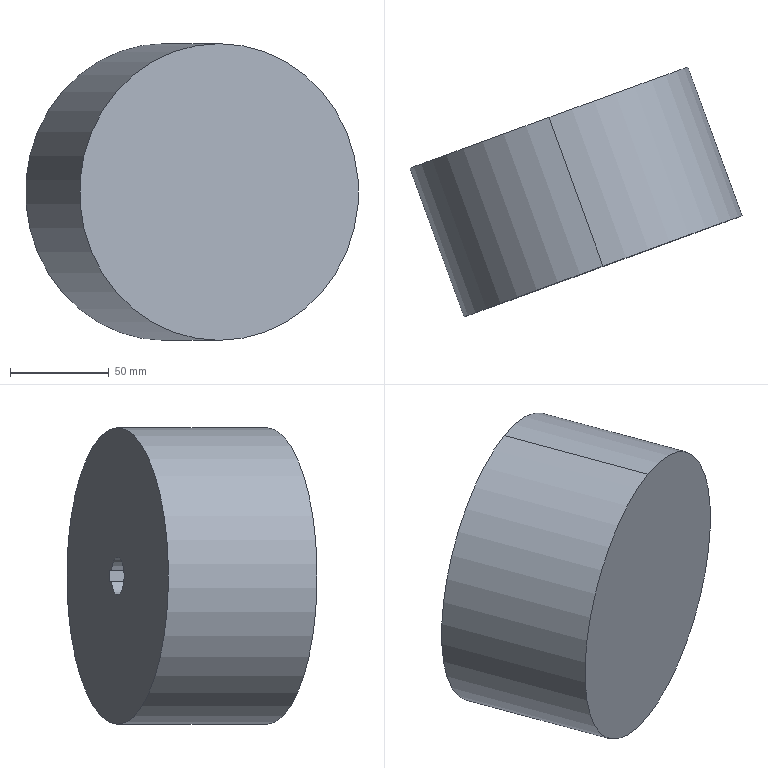Component | SolidWorks | 03-03BallDeliveryWheel-1 | 1 solid | 11 faces | box 168.32 x 126.48 x 150 mm | volume 1410704 mm3 | plane 6 | cylinder 5 | commonest cylinder face diameters 19 x3 150 x2
build123d program:
from build123d import *

# Parameters (mm, degrees)
SKETCH1_2_R         = 75
BOSS_EXTRUDE1_DEPTH = 80
CUT_EXTRUDE1_DEPTH  = 10


with BuildPart() as part:
    # Sketch1_2 → Boss-Extrude1 (new body)
    with BuildSketch(Plane(origin=(0, 0, 0), x_dir=(1, 0, 0), z_dir=(0, 1, 0))):
        with Locations(Location((0, 0, 0), (0, 0, 270))):
            Circle(SKETCH1_2_R)
    extrude(amount=BOSS_EXTRUDE1_DEPTH)

    # Sketch1 → Cut-Extrude1 (cut)
    with BuildSketch(Plane(origin=(0, 80, 0), x_dir=(1, 0, 0), z_dir=(0, 1, 0))):
        with BuildLine():
            Line((9.014, -3), (12.3, -3))
            Line((12.3, -3), (12.3, 3))
            Line((12.3, 3), (9.014, 3))
            ThreePointArc((9.014, 3), (-9.5, 0), (9.014, -3))
        make_face()
    extrude(amount=-CUT_EXTRUDE1_DEPTH, mode=Mode.SUBTRACT)


solid = part.part

# Placed as in the assembly
solid = solid.moved(Location((285.217, 218.335, 175), (0, 0, 20)))
STEP:
#1=COLOUR_RGB('',0.7922,0.8196,0.9333);
#2=FILL_AREA_STYLE_COLOUR('',#1);
#3=FILL_AREA_STYLE('',(#2));
#4=SURFACE_STYLE_FILL_AREA(#3);
#5=SURFACE_SIDE_STYLE('',(#4));
#6=SURFACE_STYLE_USAGE(.BOTH.,#5);
#7=PRESENTATION_STYLE_ASSIGNMENT((#6));
#8=CARTESIAN_POINT('',(10.286,11.186,6.516));
#9=VERTEX_POINT('',#8);
#10=CARTESIAN_POINT('',(10.286,11.186,7.264));
#11=VERTEX_POINT('',#10);
#12=CARTESIAN_POINT('',(10.286,11.186,6.89));
#13=DIRECTION('',(-0.342,0.9397,0.));
#14=DIRECTION('',(0.,0.,1.));
#15=AXIS2_PLACEMENT_3D('',#12,#13,#14);
#16=CIRCLE('',#15,0.374);
#17=EDGE_CURVE('',#9,#11,#16,.T.);
#18=ORIENTED_EDGE('',*,*,#17,.F.);
#19=CARTESIAN_POINT('',(10.152,11.556,6.516));
#20=VERTEX_POINT('',#19);
#21=CARTESIAN_POINT('',(10.286,11.186,6.516));
#22=DIRECTION('',(-0.342,0.9397,0.));
#23=VECTOR('',#22,39.37);
#24=LINE('',#21,#23);
#25=EDGE_CURVE('',#9,#20,#24,.T.);
#26=ORIENTED_EDGE('',*,*,#25,.T.);
#27=CARTESIAN_POINT('',(10.152,11.556,7.264));
#28=VERTEX_POINT('',#27);
#29=CARTESIAN_POINT('',(10.152,11.556,6.89));
#30=DIRECTION('',(-0.342,0.9397,0.));
#31=DIRECTION('',(0.,0.,1.));
#32=AXIS2_PLACEMENT_3D('',#29,#30,#31);
#33=CIRCLE('',#32,0.374);
#34=EDGE_CURVE('',#20,#28,#33,.T.);
#35=ORIENTED_EDGE('',*,*,#34,.T.);
#36=CARTESIAN_POINT('',(10.286,11.186,7.264));
#37=DIRECTION('',(-0.342,0.9397,0.));
#38=VECTOR('',#37,39.37);
#39=LINE('',#36,#38);
#40=EDGE_CURVE('',#11,#28,#39,.T.);
#41=ORIENTED_EDGE('',*,*,#40,.F.);
#42=EDGE_LOOP('',(#18,#26,#35,#41));
#43=FACE_OUTER_BOUND('',#42,.T.);
#44=CARTESIAN_POINT('',(10.286,11.186,6.89));
#45=DIRECTION('',(-0.342,0.9397,0.));
#46=DIRECTION('',(0.,0.,1.));
#47=AXIS2_PLACEMENT_3D('',#44,#45,#46);
#48=CYLINDRICAL_SURFACE('',#47,0.374);
#49=ADVANCED_FACE('',(#43),#48,.F.);
#50=CARTESIAN_POINT('',(10.62,11.307,7.008));
#51=VERTEX_POINT('',#50);
#52=CARTESIAN_POINT('',(10.286,11.186,6.89));
#53=DIRECTION('',(-0.342,0.9397,0.));
#54=DIRECTION('',(0.,0.,1.));
#55=AXIS2_PLACEMENT_3D('',#52,#53,#54);
#56=CIRCLE('',#55,0.374);
#57=EDGE_CURVE('',#11,#51,#56,.T.);
#58=ORIENTED_EDGE('',*,*,#57,.F.);
#59=ORIENTED_EDGE('',*,*,#40,.T.);
#60=CARTESIAN_POINT('',(10.485,11.677,7.008));
#61=VERTEX_POINT('',#60);
#62=CARTESIAN_POINT('',(10.152,11.556,6.89));
#63=DIRECTION('',(-0.342,0.9397,0.));
#64=DIRECTION('',(0.,0.,1.));
#65=AXIS2_PLACEMENT_3D('',#62,#63,#64);
#66=CIRCLE('',#65,0.374);
#67=EDGE_CURVE('',#28,#61,#66,.T.);
#68=ORIENTED_EDGE('',*,*,#67,.T.);
#69=CARTESIAN_POINT('',(10.62,11.307,7.008));
#70=DIRECTION('',(-0.342,0.9397,0.));
#71=VECTOR('',#70,39.37);
#72=LINE('',#69,#71);
#73=EDGE_CURVE('',#51,#61,#72,.T.);
#74=ORIENTED_EDGE('',*,*,#73,.F.);
#75=EDGE_LOOP('',(#58,#59,#68,#74));
#76=FACE_OUTER_BOUND('',#75,.T.);
#77=CARTESIAN_POINT('',(10.286,11.186,6.89));
#78=DIRECTION('',(-0.342,0.9397,0.));
#79=DIRECTION('',(0.,0.,1.));
#80=AXIS2_PLACEMENT_3D('',#77,#78,#79);
#81=CYLINDRICAL_SURFACE('',#80,0.374);
#82=ADVANCED_FACE('',(#76),#81,.F.);
#83=CARTESIAN_POINT('',(10.152,11.556,9.843));
#84=VERTEX_POINT('',#83);
#85=CARTESIAN_POINT('',(10.152,11.556,3.937));
#86=VERTEX_POINT('',#85);
#87=CARTESIAN_POINT('',(10.152,11.556,6.89));
#88=DIRECTION('',(-0.342,0.9397,0.));
#89=DIRECTION('',(0.,0.,1.));
#90=AXIS2_PLACEMENT_3D('',#87,#88,#89);
#91=CIRCLE('',#90,2.953);
#92=EDGE_CURVE('',#84,#86,#91,.T.);
#93=ORIENTED_EDGE('',*,*,#92,.F.);
#94=CARTESIAN_POINT('',(11.229,8.596,9.843));
#95=VERTEX_POINT('',#94);
#96=CARTESIAN_POINT('',(10.152,11.556,9.843));
#97=DIRECTION('',(0.342,-0.9397,-0.));
#98=VECTOR('',#97,39.37);
#99=LINE('',#96,#98);
#100=EDGE_CURVE('',#84,#95,#99,.T.);
#101=ORIENTED_EDGE('',*,*,#100,.T.);
#102=CARTESIAN_POINT('',(11.229,8.596,3.937));
#103=VERTEX_POINT('',#102);
#104=CARTESIAN_POINT('',(11.229,8.596,6.89));
#105=DIRECTION('',(-0.342,0.9397,0.));
#106=DIRECTION('',(0.,0.,1.));
#107=AXIS2_PLACEMENT_3D('',#104,#105,#106);
#108=CIRCLE('',#107,2.953);
#109=EDGE_CURVE('',#95,#103,#108,.T.);
#110=ORIENTED_EDGE('',*,*,#109,.T.);
#111=CARTESIAN_POINT('',(10.152,11.556,3.937));
#112=DIRECTION('',(0.342,-0.9397,-0.));
#113=VECTOR('',#112,39.37);
#114=LINE('',#111,#113);
#115=EDGE_CURVE('',#86,#103,#114,.T.);
#116=ORIENTED_EDGE('',*,*,#115,.F.);
#117=EDGE_LOOP('',(#93,#101,#110,#116));
#118=FACE_OUTER_BOUND('',#117,.T.);
#119=CARTESIAN_POINT('',(10.152,11.556,6.89));
#120=DIRECTION('',(0.342,-0.9397,-0.));
#121=DIRECTION('',(0.,0.,-1.));
#122=AXIS2_PLACEMENT_3D('',#119,#120,#121);
#123=CYLINDRICAL_SURFACE('',#122,2.953);
#124=ADVANCED_FACE('',(#118),#123,.T.);
#125=ORIENTED_EDGE('',*,*,#100,.F.);
#126=CARTESIAN_POINT('',(10.152,11.556,6.89));
#127=DIRECTION('',(-0.342,0.9397,0.));
#128=DIRECTION('',(0.,0.,1.));
#129=AXIS2_PLACEMENT_3D('',#126,#127,#128);
#130=CIRCLE('',#129,2.953);
#131=EDGE_CURVE('',#86,#84,#130,.T.);
#132=ORIENTED_EDGE('',*,*,#131,.F.);
#133=ORIENTED_EDGE('',*,*,#115,.T.);
#134=CARTESIAN_POINT('',(11.229,8.596,6.89));
#135=DIRECTION('',(-0.342,0.9397,0.));
#136=DIRECTION('',(0.,0.,1.));
#137=AXIS2_PLACEMENT_3D('',#134,#135,#136);
#138=CIRCLE('',#137,2.953);
#139=EDGE_CURVE('',#103,#95,#138,.T.);
#140=ORIENTED_EDGE('',*,*,#139,.T.);
#141=EDGE_LOOP('',(#125,#132,#133,#140));
#142=FACE_OUTER_BOUND('',#141,.T.);
#143=CARTESIAN_POINT('',(10.152,11.556,6.89));
#144=DIRECTION('',(0.342,-0.9397,-0.));
#145=DIRECTION('',(0.,0.,-1.));
#146=AXIS2_PLACEMENT_3D('',#143,#144,#145);
#147=CYLINDRICAL_SURFACE('',#146,2.953);
#148=ADVANCED_FACE('',(#142),#147,.T.);
#149=CARTESIAN_POINT('',(10.485,11.677,6.772));
#150=VERTEX_POINT('',#149);
#151=CARTESIAN_POINT('',(10.152,11.556,6.89));
#152=DIRECTION('',(-0.342,0.9397,0.));
#153=DIRECTION('',(0.,0.,1.));
#154=AXIS2_PLACEMENT_3D('',#151,#152,#153);
#155=CIRCLE('',#154,0.374);
#156=EDGE_CURVE('',#150,#20,#155,.T.);
#157=ORIENTED_EDGE('',*,*,#156,.F.);
#158=CARTESIAN_POINT('',(10.607,11.721,6.772));
#159=VERTEX_POINT('',#158);
#160=CARTESIAN_POINT('',(10.607,11.721,6.772));
#161=DIRECTION('',(-0.9397,-0.342,0.));
#162=VECTOR('',#161,39.37);
#163=LINE('',#160,#162);
#164=EDGE_CURVE('',#159,#150,#163,.T.);
#165=ORIENTED_EDGE('',*,*,#164,.F.);
#166=CARTESIAN_POINT('',(10.607,11.721,7.008));
#167=VERTEX_POINT('',#166);
#168=CARTESIAN_POINT('',(10.607,11.721,7.008));
#169=DIRECTION('',(-0.,0.,-1.));
#170=VECTOR('',#169,39.37);
#171=LINE('',#168,#170);
#172=EDGE_CURVE('',#167,#159,#171,.T.);
#173=ORIENTED_EDGE('',*,*,#172,.F.);
#174=CARTESIAN_POINT('',(10.485,11.677,7.008));
#175=DIRECTION('',(0.9397,0.342,0.));
#176=VECTOR('',#175,39.37);
#177=LINE('',#174,#176);
#178=EDGE_CURVE('',#61,#167,#177,.T.);
#179=ORIENTED_EDGE('',*,*,#178,.F.);
#180=ORIENTED_EDGE('',*,*,#67,.F.);
#181=ORIENTED_EDGE('',*,*,#34,.F.);
#182=EDGE_LOOP('',(#157,#165,#173,#179,#180,#181));
#183=FACE_BOUND('',#182,.T.);
#184=ORIENTED_EDGE('',*,*,#131,.T.);
#185=ORIENTED_EDGE('',*,*,#92,.T.);
#186=EDGE_LOOP('',(#184,#185));
#187=FACE_OUTER_BOUND('',#186,.T.);
#188=CARTESIAN_POINT('',(10.152,11.556,6.89));
#189=DIRECTION('',(-0.342,0.9397,0.));
#190=DIRECTION('',(0.,-0.,1.));
#191=AXIS2_PLACEMENT_3D('',#188,#189,#190);
#192=PLANE('',#191);
#193=ADVANCED_FACE('',(#183,#187),#192,.T.);
#194=ORIENTED_EDGE('',*,*,#139,.F.);
#195=ORIENTED_EDGE('',*,*,#109,.F.);
#196=EDGE_LOOP('',(#194,#195));
#197=FACE_OUTER_BOUND('',#196,.T.);
#198=CARTESIAN_POINT('',(11.229,8.596,6.89));
#199=DIRECTION('',(-0.342,0.9397,0.));
#200=DIRECTION('',(0.,-0.,1.));
#201=AXIS2_PLACEMENT_3D('',#198,#199,#200);
#202=PLANE('',#201);
#203=ADVANCED_FACE('',(#197),#202,.F.);
#204=ORIENTED_EDGE('',*,*,#25,.F.);
#205=CARTESIAN_POINT('',(10.62,11.307,6.772));
#206=VERTEX_POINT('',#205);
#207=CARTESIAN_POINT('',(10.286,11.186,6.89));
#208=DIRECTION('',(-0.342,0.9397,0.));
#209=DIRECTION('',(0.,0.,1.));
#210=AXIS2_PLACEMENT_3D('',#207,#208,#209);
#211=CIRCLE('',#210,0.374);
#212=EDGE_CURVE('',#206,#9,#211,.T.);
#213=ORIENTED_EDGE('',*,*,#212,.F.);
#214=CARTESIAN_POINT('',(10.62,11.307,6.772));
#215=DIRECTION('',(-0.342,0.9397,0.));
#216=VECTOR('',#215,39.37);
#217=LINE('',#214,#216);
#218=EDGE_CURVE('',#206,#150,#217,.T.);
#219=ORIENTED_EDGE('',*,*,#218,.T.);
#220=ORIENTED_EDGE('',*,*,#156,.T.);
#221=EDGE_LOOP('',(#204,#213,#219,#220));
#222=FACE_OUTER_BOUND('',#221,.T.);
#223=CARTESIAN_POINT('',(10.286,11.186,6.89));
#224=DIRECTION('',(-0.342,0.9397,0.));
#225=DIRECTION('',(0.,0.,1.));
#226=AXIS2_PLACEMENT_3D('',#223,#224,#225);
#227=CYLINDRICAL_SURFACE('',#226,0.374);
#228=ADVANCED_FACE('',(#222),#227,.F.);
#229=ORIENTED_EDGE('',*,*,#164,.T.);
#230=ORIENTED_EDGE('',*,*,#218,.F.);
#231=CARTESIAN_POINT('',(10.741,11.351,6.772));
#232=VERTEX_POINT('',#231);
#233=CARTESIAN_POINT('',(10.741,11.351,6.772));
#234=DIRECTION('',(-0.9397,-0.342,0.));
#235=VECTOR('',#234,39.37);
#236=LINE('',#233,#235);
#237=EDGE_CURVE('',#232,#206,#236,.T.);
#238=ORIENTED_EDGE('',*,*,#237,.F.);
#239=CARTESIAN_POINT('',(10.741,11.351,6.772));
#240=DIRECTION('',(-0.342,0.9397,0.));
#241=VECTOR('',#240,39.37);
#242=LINE('',#239,#241);
#243=EDGE_CURVE('',#232,#159,#242,.T.);
#244=ORIENTED_EDGE('',*,*,#243,.T.);
#245=EDGE_LOOP('',(#229,#230,#238,#244));
#246=FACE_OUTER_BOUND('',#245,.T.);
#247=CARTESIAN_POINT('',(10.741,11.351,6.772));
#248=DIRECTION('',(-0.,0.,-1.));
#249=DIRECTION('',(-0.9397,-0.342,0.));
#250=AXIS2_PLACEMENT_3D('',#247,#248,#249);
#251=PLANE('',#250);
#252=ADVANCED_FACE('',(#246),#251,.F.);
#253=ORIENTED_EDGE('',*,*,#172,.T.);
#254=ORIENTED_EDGE('',*,*,#243,.F.);
#255=CARTESIAN_POINT('',(10.741,11.351,7.008));
#256=VERTEX_POINT('',#255);
#257=CARTESIAN_POINT('',(10.741,11.351,7.008));
#258=DIRECTION('',(-0.,0.,-1.));
#259=VECTOR('',#258,39.37);
#260=LINE('',#257,#259);
#261=EDGE_CURVE('',#256,#232,#260,.T.);
#262=ORIENTED_EDGE('',*,*,#261,.F.);
#263=CARTESIAN_POINT('',(10.741,11.351,7.008));
#264=DIRECTION('',(-0.342,0.9397,0.));
#265=VECTOR('',#264,39.37);
#266=LINE('',#263,#265);
#267=EDGE_CURVE('',#256,#167,#266,.T.);
#268=ORIENTED_EDGE('',*,*,#267,.T.);
#269=EDGE_LOOP('',(#253,#254,#262,#268));
#270=FACE_OUTER_BOUND('',#269,.T.);
#271=CARTESIAN_POINT('',(10.741,11.351,7.008));
#272=DIRECTION('',(0.9397,0.342,0.));
#273=DIRECTION('',(-0.,0.,-1.));
#274=AXIS2_PLACEMENT_3D('',#271,#272,#273);
#275=PLANE('',#274);
#276=ADVANCED_FACE('',(#270),#275,.F.);
#277=ORIENTED_EDGE('',*,*,#178,.T.);
#278=ORIENTED_EDGE('',*,*,#267,.F.);
#279=CARTESIAN_POINT('',(10.62,11.307,7.008));
#280=DIRECTION('',(0.9397,0.342,0.));
#281=VECTOR('',#280,39.37);
#282=LINE('',#279,#281);
#283=EDGE_CURVE('',#51,#256,#282,.T.);
#284=ORIENTED_EDGE('',*,*,#283,.F.);
#285=ORIENTED_EDGE('',*,*,#73,.T.);
#286=EDGE_LOOP('',(#277,#278,#284,#285));
#287=FACE_OUTER_BOUND('',#286,.T.);
#288=CARTESIAN_POINT('',(10.62,11.307,7.008));
#289=DIRECTION('',(0.,-0.,1.));
#290=DIRECTION('',(0.9397,0.342,0.));
#291=AXIS2_PLACEMENT_3D('',#288,#289,#290);
#292=PLANE('',#291);
#293=ADVANCED_FACE('',(#287),#292,.F.);
#294=ORIENTED_EDGE('',*,*,#212,.T.);
#295=ORIENTED_EDGE('',*,*,#17,.T.);
#296=ORIENTED_EDGE('',*,*,#57,.T.);
#297=ORIENTED_EDGE('',*,*,#283,.T.);
#298=ORIENTED_EDGE('',*,*,#261,.T.);
#299=ORIENTED_EDGE('',*,*,#237,.T.);
#300=EDGE_LOOP('',(#294,#295,#296,#297,#298,#299));
#301=FACE_OUTER_BOUND('',#300,.T.);
#302=CARTESIAN_POINT('',(10.286,11.186,6.89));
#303=DIRECTION('',(-0.342,0.9397,0.));
#304=DIRECTION('',(0.,-0.,1.));
#305=AXIS2_PLACEMENT_3D('',#302,#303,#304);
#306=PLANE('',#305);
#307=ADVANCED_FACE('',(#301),#306,.T.);
#308=CLOSED_SHELL('',(#49,#82,#124,#148,#193,#203,#228,#252,#276,#293,#307));
#309=MANIFOLD_SOLID_BREP('',#308);
#310=STYLED_ITEM('',(#7),#309);
#311=(LENGTH_UNIT()NAMED_UNIT(*)SI_UNIT($,.METRE.));
#312=LENGTH_MEASURE_WITH_UNIT(LENGTH_MEASURE(0.0254),#311);
#313=DIMENSIONAL_EXPONENTS(1.,0.,0.,0.,0.,0.,0.);
#314=(CONVERSION_BASED_UNIT('',#312)LENGTH_UNIT()NAMED_UNIT(#313));
#315=UNCERTAINTY_MEASURE_WITH_UNIT(LENGTH_MEASURE(0.00001),#314,'','');
#316=(NAMED_UNIT(*)PLANE_ANGLE_UNIT()SI_UNIT($,.RADIAN.));
#317=(NAMED_UNIT(*)SI_UNIT($,.STERADIAN.)SOLID_ANGLE_UNIT());
#318=(GEOMETRIC_REPRESENTATION_CONTEXT(3)GLOBAL_UNCERTAINTY_ASSIGNED_CONTEXT((#315))GLOBAL_UNIT_ASSIGNED_CONTEXT((#314,#316,#317))REPRESENTATION_CONTEXT('',''));
#319=MECHANICAL_DESIGN_GEOMETRIC_PRESENTATION_REPRESENTATION('',(#310),#318);
#320=PRESENTATION_LAYER_ASSIGNMENT('','',(#310));
#321=CARTESIAN_POINT('',(0.,0.,0.));
#322=DIRECTION('',(0.,0.,1.));
#323=DIRECTION('',(1.,0.,0.));
#324=AXIS2_PLACEMENT_3D('',#321,#322,#323);
#325=(LENGTH_UNIT()NAMED_UNIT(*)SI_UNIT($,.METRE.));
#326=LENGTH_MEASURE_WITH_UNIT(LENGTH_MEASURE(0.0254),#325);
#327=DIMENSIONAL_EXPONENTS(1.,0.,0.,0.,0.,0.,0.);
#328=(CONVERSION_BASED_UNIT('',#326)LENGTH_UNIT()NAMED_UNIT(#327));
#329=UNCERTAINTY_MEASURE_WITH_UNIT(LENGTH_MEASURE(0.00001),#328,'','');
#330=(NAMED_UNIT(*)PLANE_ANGLE_UNIT()SI_UNIT($,.RADIAN.));
#331=(NAMED_UNIT(*)SI_UNIT($,.STERADIAN.)SOLID_ANGLE_UNIT());
#332=(GEOMETRIC_REPRESENTATION_CONTEXT(3)GLOBAL_UNCERTAINTY_ASSIGNED_CONTEXT((#329))GLOBAL_UNIT_ASSIGNED_CONTEXT((#328,#330,#331))REPRESENTATION_CONTEXT('',''));
#333=ADVANCED_BREP_SHAPE_REPRESENTATION('',(#309,#324),#332);